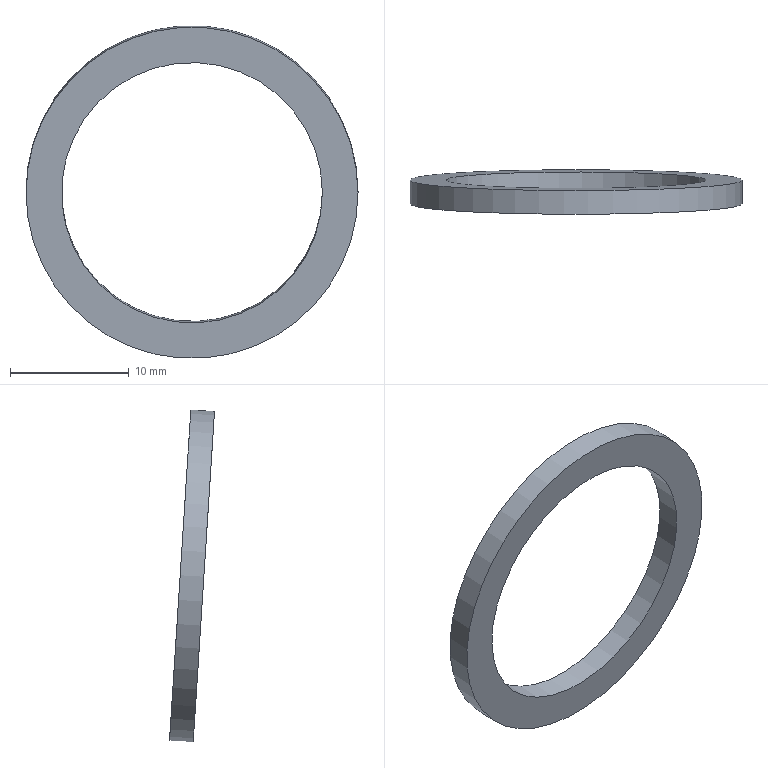Component | NX | CCJ-015 | 1 solid | 4 faces | box 28 x 3.8 x 28.07 mm | volume 471 mm3 | plane 2 | cylinder 2 | commonest cylinder face diameters 28 x1 22 x1
STEP:
#1=CARTESIAN_POINT('',(0.,0.,0.));
#2=DIRECTION('',(0.,0.,1.));
#3=DIRECTION('',(1.,0.,0.));
#4=AXIS2_PLACEMENT_3D('',#1,#2,#3);
#5=CARTESIAN_POINT('',(39.,-8.106,192.909));
#6=VERTEX_POINT('',#5);
#7=CARTESIAN_POINT('',(25.,-8.106,192.909));
#8=DIRECTION('',(0.,0.9979,0.06443));
#9=DIRECTION('',(1.,0.,0.));
#10=AXIS2_PLACEMENT_3D('',#7,#8,#9);
#11=CIRCLE('',#10,14.);
#12=CARTESIAN_POINT('',(25.,-8.106,192.909));
#13=DIRECTION('',(0.,-0.9979,-0.06443));
#14=DIRECTION('',(-1.,0.,0.));
#15=AXIS2_PLACEMENT_3D('',#12,#13,#14);
#16=PLANE('',#15);
#17=CARTESIAN_POINT('',(-14.,0.));
#18=CARTESIAN_POINT('',(-14.,24.249));
#19=CARTESIAN_POINT('',(7.,12.124));
#20=CARTESIAN_POINT('',(28.,0.));
#21=CARTESIAN_POINT('',(7.,-12.124));
#22=CARTESIAN_POINT('',(-14.,-24.249));
#23=CARTESIAN_POINT('',(-14.,0.));
#24=(BOUNDED_CURVE()B_SPLINE_CURVE(2,(#17,#18,#19,#20,#21,#22,#23),.UNSPECIFIED.,.T.,.F.)B_SPLINE_CURVE_WITH_KNOTS((1,2,2,2,2,1),(-2.094,0.,2.094,4.189,6.283,8.378),.UNSPECIFIED.)CURVE()GEOMETRIC_REPRESENTATION_ITEM()RATIONAL_B_SPLINE_CURVE((1.,0.5,1.,0.5,1.,0.5,1.))REPRESENTATION_ITEM(''));
#25=(GEOMETRIC_REPRESENTATION_CONTEXT(2)PARAMETRIC_REPRESENTATION_CONTEXT()REPRESENTATION_CONTEXT('',''));
#26=DEFINITIONAL_REPRESENTATION('',(#24),#25);
#27=PCURVE('',#16,#26);
#28=CARTESIAN_POINT('',(25.,-8.106,192.909));
#29=DIRECTION('',(0.,0.9979,0.06443));
#30=DIRECTION('',(1.,0.,0.));
#31=AXIS2_PLACEMENT_3D('',#28,#29,#30);
#32=CYLINDRICAL_SURFACE('',#31,14.);
#33=CARTESIAN_POINT('',(0.,0.));
#34=DIRECTION('',(1.,0.));
#35=VECTOR('',#34,1.);
#36=LINE('',#33,#35);
#37=(GEOMETRIC_REPRESENTATION_CONTEXT(2)PARAMETRIC_REPRESENTATION_CONTEXT()REPRESENTATION_CONTEXT('',''));
#38=DEFINITIONAL_REPRESENTATION('',(#36),#37);
#39=PCURVE('',#32,#38);
#40=SURFACE_CURVE('',#11,(#27,#39),.PCURVE_S1.);
#41=EDGE_CURVE('',#6,#6,#40,.T.);
#42=ORIENTED_EDGE('',*,*,#41,.F.);
#43=EDGE_LOOP('',(#42));
#44=FACE_BOUND('',#43,.T.);
#45=CARTESIAN_POINT('',(36.,-8.106,192.909));
#46=VERTEX_POINT('',#45);
#47=CARTESIAN_POINT('',(25.,-8.106,192.909));
#48=DIRECTION('',(0.,0.9979,0.06443));
#49=DIRECTION('',(1.,0.,0.));
#50=AXIS2_PLACEMENT_3D('',#47,#48,#49);
#51=CIRCLE('',#50,11.);
#52=CARTESIAN_POINT('',(-11.,0.));
#53=CARTESIAN_POINT('',(-11.,19.053));
#54=CARTESIAN_POINT('',(5.5,9.526));
#55=CARTESIAN_POINT('',(22.,0.));
#56=CARTESIAN_POINT('',(5.5,-9.526));
#57=CARTESIAN_POINT('',(-11.,-19.053));
#58=CARTESIAN_POINT('',(-11.,0.));
#59=(BOUNDED_CURVE()B_SPLINE_CURVE(2,(#52,#53,#54,#55,#56,#57,#58),.UNSPECIFIED.,.T.,.F.)B_SPLINE_CURVE_WITH_KNOTS((1,2,2,2,2,1),(-2.094,0.,2.094,4.189,6.283,8.378),.UNSPECIFIED.)CURVE()GEOMETRIC_REPRESENTATION_ITEM()RATIONAL_B_SPLINE_CURVE((1.,0.5,1.,0.5,1.,0.5,1.))REPRESENTATION_ITEM(''));
#60=(GEOMETRIC_REPRESENTATION_CONTEXT(2)PARAMETRIC_REPRESENTATION_CONTEXT()REPRESENTATION_CONTEXT('',''));
#61=DEFINITIONAL_REPRESENTATION('',(#59),#60);
#62=PCURVE('',#16,#61);
#63=CARTESIAN_POINT('',(25.,-8.106,192.909));
#64=DIRECTION('',(0.,0.9979,0.06443));
#65=DIRECTION('',(1.,0.,0.));
#66=AXIS2_PLACEMENT_3D('',#63,#64,#65);
#67=CYLINDRICAL_SURFACE('',#66,11.);
#68=CARTESIAN_POINT('',(0.,0.));
#69=DIRECTION('',(1.,0.));
#70=VECTOR('',#69,1.);
#71=LINE('',#68,#70);
#72=(GEOMETRIC_REPRESENTATION_CONTEXT(2)PARAMETRIC_REPRESENTATION_CONTEXT()REPRESENTATION_CONTEXT('',''));
#73=DEFINITIONAL_REPRESENTATION('',(#71),#72);
#74=PCURVE('',#67,#73);
#75=SURFACE_CURVE('',#51,(#62,#74),.PCURVE_S1.);
#76=EDGE_CURVE('',#46,#46,#75,.T.);
#77=ORIENTED_EDGE('',*,*,#76,.T.);
#78=EDGE_LOOP('',(#77));
#79=FACE_BOUND('',#78,.T.);
#80=ADVANCED_FACE('',(#44,#79),#16,.T.);
#81=CARTESIAN_POINT('',(39.,-6.11,193.038));
#82=VERTEX_POINT('',#81);
#83=CARTESIAN_POINT('',(25.,-6.11,193.038));
#84=DIRECTION('',(0.,0.9979,0.06443));
#85=DIRECTION('',(1.,0.,0.));
#86=AXIS2_PLACEMENT_3D('',#83,#84,#85);
#87=CIRCLE('',#86,14.);
#88=CARTESIAN_POINT('',(25.,-6.11,193.038));
#89=DIRECTION('',(0.,-0.9979,-0.06443));
#90=DIRECTION('',(-1.,0.,0.));
#91=AXIS2_PLACEMENT_3D('',#88,#89,#90);
#92=PLANE('',#91);
#93=CARTESIAN_POINT('',(-14.,0.));
#94=CARTESIAN_POINT('',(-14.,24.249));
#95=CARTESIAN_POINT('',(7.,12.124));
#96=CARTESIAN_POINT('',(28.,0.));
#97=CARTESIAN_POINT('',(7.,-12.124));
#98=CARTESIAN_POINT('',(-14.,-24.249));
#99=CARTESIAN_POINT('',(-14.,0.));
#100=(BOUNDED_CURVE()B_SPLINE_CURVE(2,(#93,#94,#95,#96,#97,#98,#99),.UNSPECIFIED.,.T.,.F.)B_SPLINE_CURVE_WITH_KNOTS((1,2,2,2,2,1),(-2.094,0.,2.094,4.189,6.283,8.378),.UNSPECIFIED.)CURVE()GEOMETRIC_REPRESENTATION_ITEM()RATIONAL_B_SPLINE_CURVE((1.,0.5,1.,0.5,1.,0.5,1.))REPRESENTATION_ITEM(''));
#101=(GEOMETRIC_REPRESENTATION_CONTEXT(2)PARAMETRIC_REPRESENTATION_CONTEXT()REPRESENTATION_CONTEXT('',''));
#102=DEFINITIONAL_REPRESENTATION('',(#100),#101);
#103=PCURVE('',#92,#102);
#104=CARTESIAN_POINT('',(0.,2.));
#105=DIRECTION('',(1.,0.));
#106=VECTOR('',#105,1.);
#107=LINE('',#104,#106);
#108=(GEOMETRIC_REPRESENTATION_CONTEXT(2)PARAMETRIC_REPRESENTATION_CONTEXT()REPRESENTATION_CONTEXT('',''));
#109=DEFINITIONAL_REPRESENTATION('',(#107),#108);
#110=PCURVE('',#32,#109);
#111=SURFACE_CURVE('',#87,(#103,#110),.PCURVE_S1.);
#112=EDGE_CURVE('',#82,#82,#111,.T.);
#113=ORIENTED_EDGE('',*,*,#112,.T.);
#114=EDGE_LOOP('',(#113));
#115=FACE_BOUND('',#114,.T.);
#116=CARTESIAN_POINT('',(36.,-6.11,193.038));
#117=VERTEX_POINT('',#116);
#118=CARTESIAN_POINT('',(25.,-6.11,193.038));
#119=DIRECTION('',(0.,0.9979,0.06443));
#120=DIRECTION('',(1.,0.,0.));
#121=AXIS2_PLACEMENT_3D('',#118,#119,#120);
#122=CIRCLE('',#121,11.);
#123=CARTESIAN_POINT('',(-11.,0.));
#124=CARTESIAN_POINT('',(-11.,19.053));
#125=CARTESIAN_POINT('',(5.5,9.526));
#126=CARTESIAN_POINT('',(22.,0.));
#127=CARTESIAN_POINT('',(5.5,-9.526));
#128=CARTESIAN_POINT('',(-11.,-19.053));
#129=CARTESIAN_POINT('',(-11.,0.));
#130=(BOUNDED_CURVE()B_SPLINE_CURVE(2,(#123,#124,#125,#126,#127,#128,#129),.UNSPECIFIED.,.T.,.F.)B_SPLINE_CURVE_WITH_KNOTS((1,2,2,2,2,1),(-2.094,0.,2.094,4.189,6.283,8.378),.UNSPECIFIED.)CURVE()GEOMETRIC_REPRESENTATION_ITEM()RATIONAL_B_SPLINE_CURVE((1.,0.5,1.,0.5,1.,0.5,1.))REPRESENTATION_ITEM(''));
#131=(GEOMETRIC_REPRESENTATION_CONTEXT(2)PARAMETRIC_REPRESENTATION_CONTEXT()REPRESENTATION_CONTEXT('',''));
#132=DEFINITIONAL_REPRESENTATION('',(#130),#131);
#133=PCURVE('',#92,#132);
#134=CARTESIAN_POINT('',(0.,2.));
#135=DIRECTION('',(1.,0.));
#136=VECTOR('',#135,1.);
#137=LINE('',#134,#136);
#138=(GEOMETRIC_REPRESENTATION_CONTEXT(2)PARAMETRIC_REPRESENTATION_CONTEXT()REPRESENTATION_CONTEXT('',''));
#139=DEFINITIONAL_REPRESENTATION('',(#137),#138);
#140=PCURVE('',#67,#139);
#141=SURFACE_CURVE('',#122,(#133,#140),.PCURVE_S1.);
#142=EDGE_CURVE('',#117,#117,#141,.T.);
#143=ORIENTED_EDGE('',*,*,#142,.F.);
#144=EDGE_LOOP('',(#143));
#145=FACE_BOUND('',#144,.T.);
#146=ADVANCED_FACE('',(#115,#145),#92,.F.);
#147=ORIENTED_EDGE('',*,*,#41,.T.);
#148=CARTESIAN_POINT('',(39.,-8.106,192.909));
#149=CARTESIAN_POINT('',(39.,-6.11,193.038));
#150=B_SPLINE_CURVE_WITH_KNOTS('',1,(#148,#149),.UNSPECIFIED.,.F.,.F.,(2,2),(0.,2.),.PIECEWISE_BEZIER_KNOTS.);
#151=CARTESIAN_POINT('',(6.283,0.));
#152=DIRECTION('',(0.,1.));
#153=VECTOR('',#152,1.);
#154=LINE('',#151,#153);
#155=(GEOMETRIC_REPRESENTATION_CONTEXT(2)PARAMETRIC_REPRESENTATION_CONTEXT()REPRESENTATION_CONTEXT('',''));
#156=DEFINITIONAL_REPRESENTATION('',(#154),#155);
#157=PCURVE('',#32,#156);
#158=CARTESIAN_POINT('',(0.,0.));
#159=DIRECTION('',(0.,1.));
#160=VECTOR('',#159,1.);
#161=LINE('',#158,#160);
#162=(GEOMETRIC_REPRESENTATION_CONTEXT(2)PARAMETRIC_REPRESENTATION_CONTEXT()REPRESENTATION_CONTEXT('',''));
#163=DEFINITIONAL_REPRESENTATION('',(#161),#162);
#164=PCURVE('',#32,#163);
#165=SEAM_CURVE('',#150,(#157,#164),.PCURVE_S1.);
#166=EDGE_CURVE('',#6,#82,#165,.T.);
#167=ORIENTED_EDGE('',*,*,#166,.T.);
#168=ORIENTED_EDGE('',*,*,#112,.F.);
#169=ORIENTED_EDGE('',*,*,#166,.F.);
#170=EDGE_LOOP('',(#147,#167,#168,#169));
#171=FACE_BOUND('',#170,.T.);
#172=ADVANCED_FACE('',(#171),#32,.T.);
#173=ORIENTED_EDGE('',*,*,#76,.T.);
#174=CARTESIAN_POINT('',(36.,-8.106,192.909));
#175=CARTESIAN_POINT('',(36.,-6.11,193.038));
#176=B_SPLINE_CURVE_WITH_KNOTS('',1,(#174,#175),.UNSPECIFIED.,.F.,.F.,(2,2),(0.,2.),.PIECEWISE_BEZIER_KNOTS.);
#177=CARTESIAN_POINT('',(6.283,0.));
#178=DIRECTION('',(0.,1.));
#179=VECTOR('',#178,1.);
#180=LINE('',#177,#179);
#181=(GEOMETRIC_REPRESENTATION_CONTEXT(2)PARAMETRIC_REPRESENTATION_CONTEXT()REPRESENTATION_CONTEXT('',''));
#182=DEFINITIONAL_REPRESENTATION('',(#180),#181);
#183=PCURVE('',#67,#182);
#184=CARTESIAN_POINT('',(0.,0.));
#185=DIRECTION('',(0.,1.));
#186=VECTOR('',#185,1.);
#187=LINE('',#184,#186);
#188=(GEOMETRIC_REPRESENTATION_CONTEXT(2)PARAMETRIC_REPRESENTATION_CONTEXT()REPRESENTATION_CONTEXT('',''));
#189=DEFINITIONAL_REPRESENTATION('',(#187),#188);
#190=PCURVE('',#67,#189);
#191=SEAM_CURVE('',#176,(#183,#190),.PCURVE_S1.);
#192=EDGE_CURVE('',#46,#117,#191,.T.);
#193=ORIENTED_EDGE('',*,*,#192,.T.);
#194=ORIENTED_EDGE('',*,*,#142,.F.);
#195=ORIENTED_EDGE('',*,*,#192,.F.);
#196=EDGE_LOOP('',(#173,#193,#194,#195));
#197=FACE_BOUND('',#196,.F.);
#198=ADVANCED_FACE('',(#197),#67,.F.);
#199=CLOSED_SHELL('',(#80,#146,#172,#198));
#200=MANIFOLD_SOLID_BREP('',#199);
#201=(LENGTH_UNIT()NAMED_UNIT(*)SI_UNIT(.MILLI.,.METRE.));
#202=UNCERTAINTY_MEASURE_WITH_UNIT(LENGTH_MEASURE(0.00001),#201,'','');
#203=(NAMED_UNIT(*)PLANE_ANGLE_UNIT()SI_UNIT($,.RADIAN.));
#204=(NAMED_UNIT(*)SI_UNIT($,.STERADIAN.)SOLID_ANGLE_UNIT());
#205=(GEOMETRIC_REPRESENTATION_CONTEXT(3)GLOBAL_UNCERTAINTY_ASSIGNED_CONTEXT((#202))GLOBAL_UNIT_ASSIGNED_CONTEXT((#201,#203,#204))REPRESENTATION_CONTEXT('',''));
#206=ADVANCED_BREP_SHAPE_REPRESENTATION('',(#4,#200),#205);